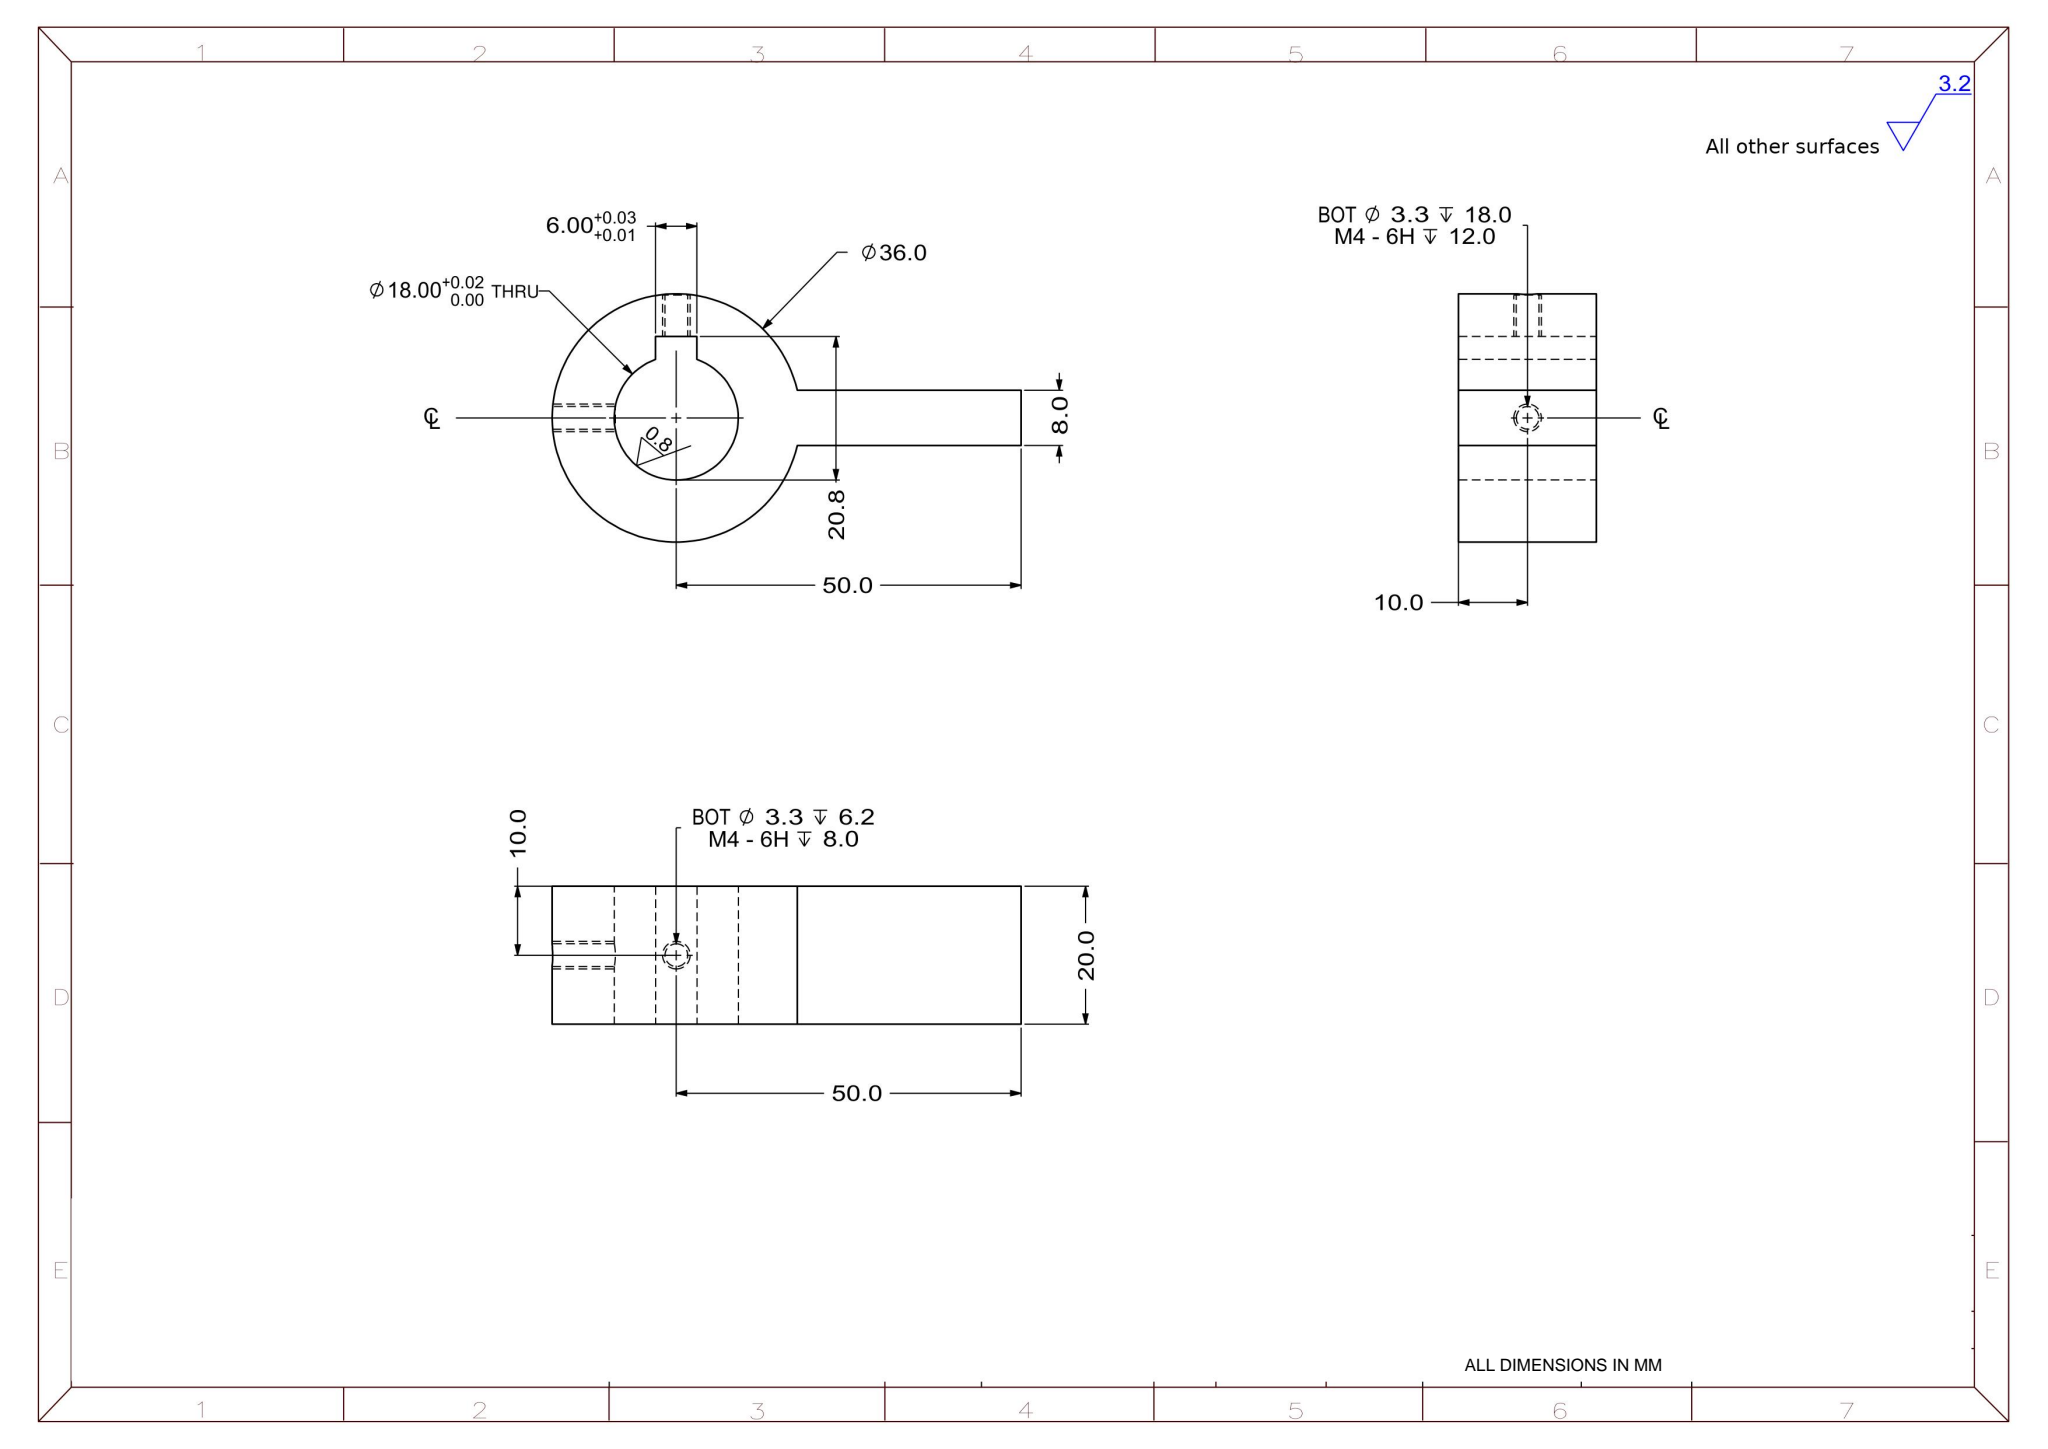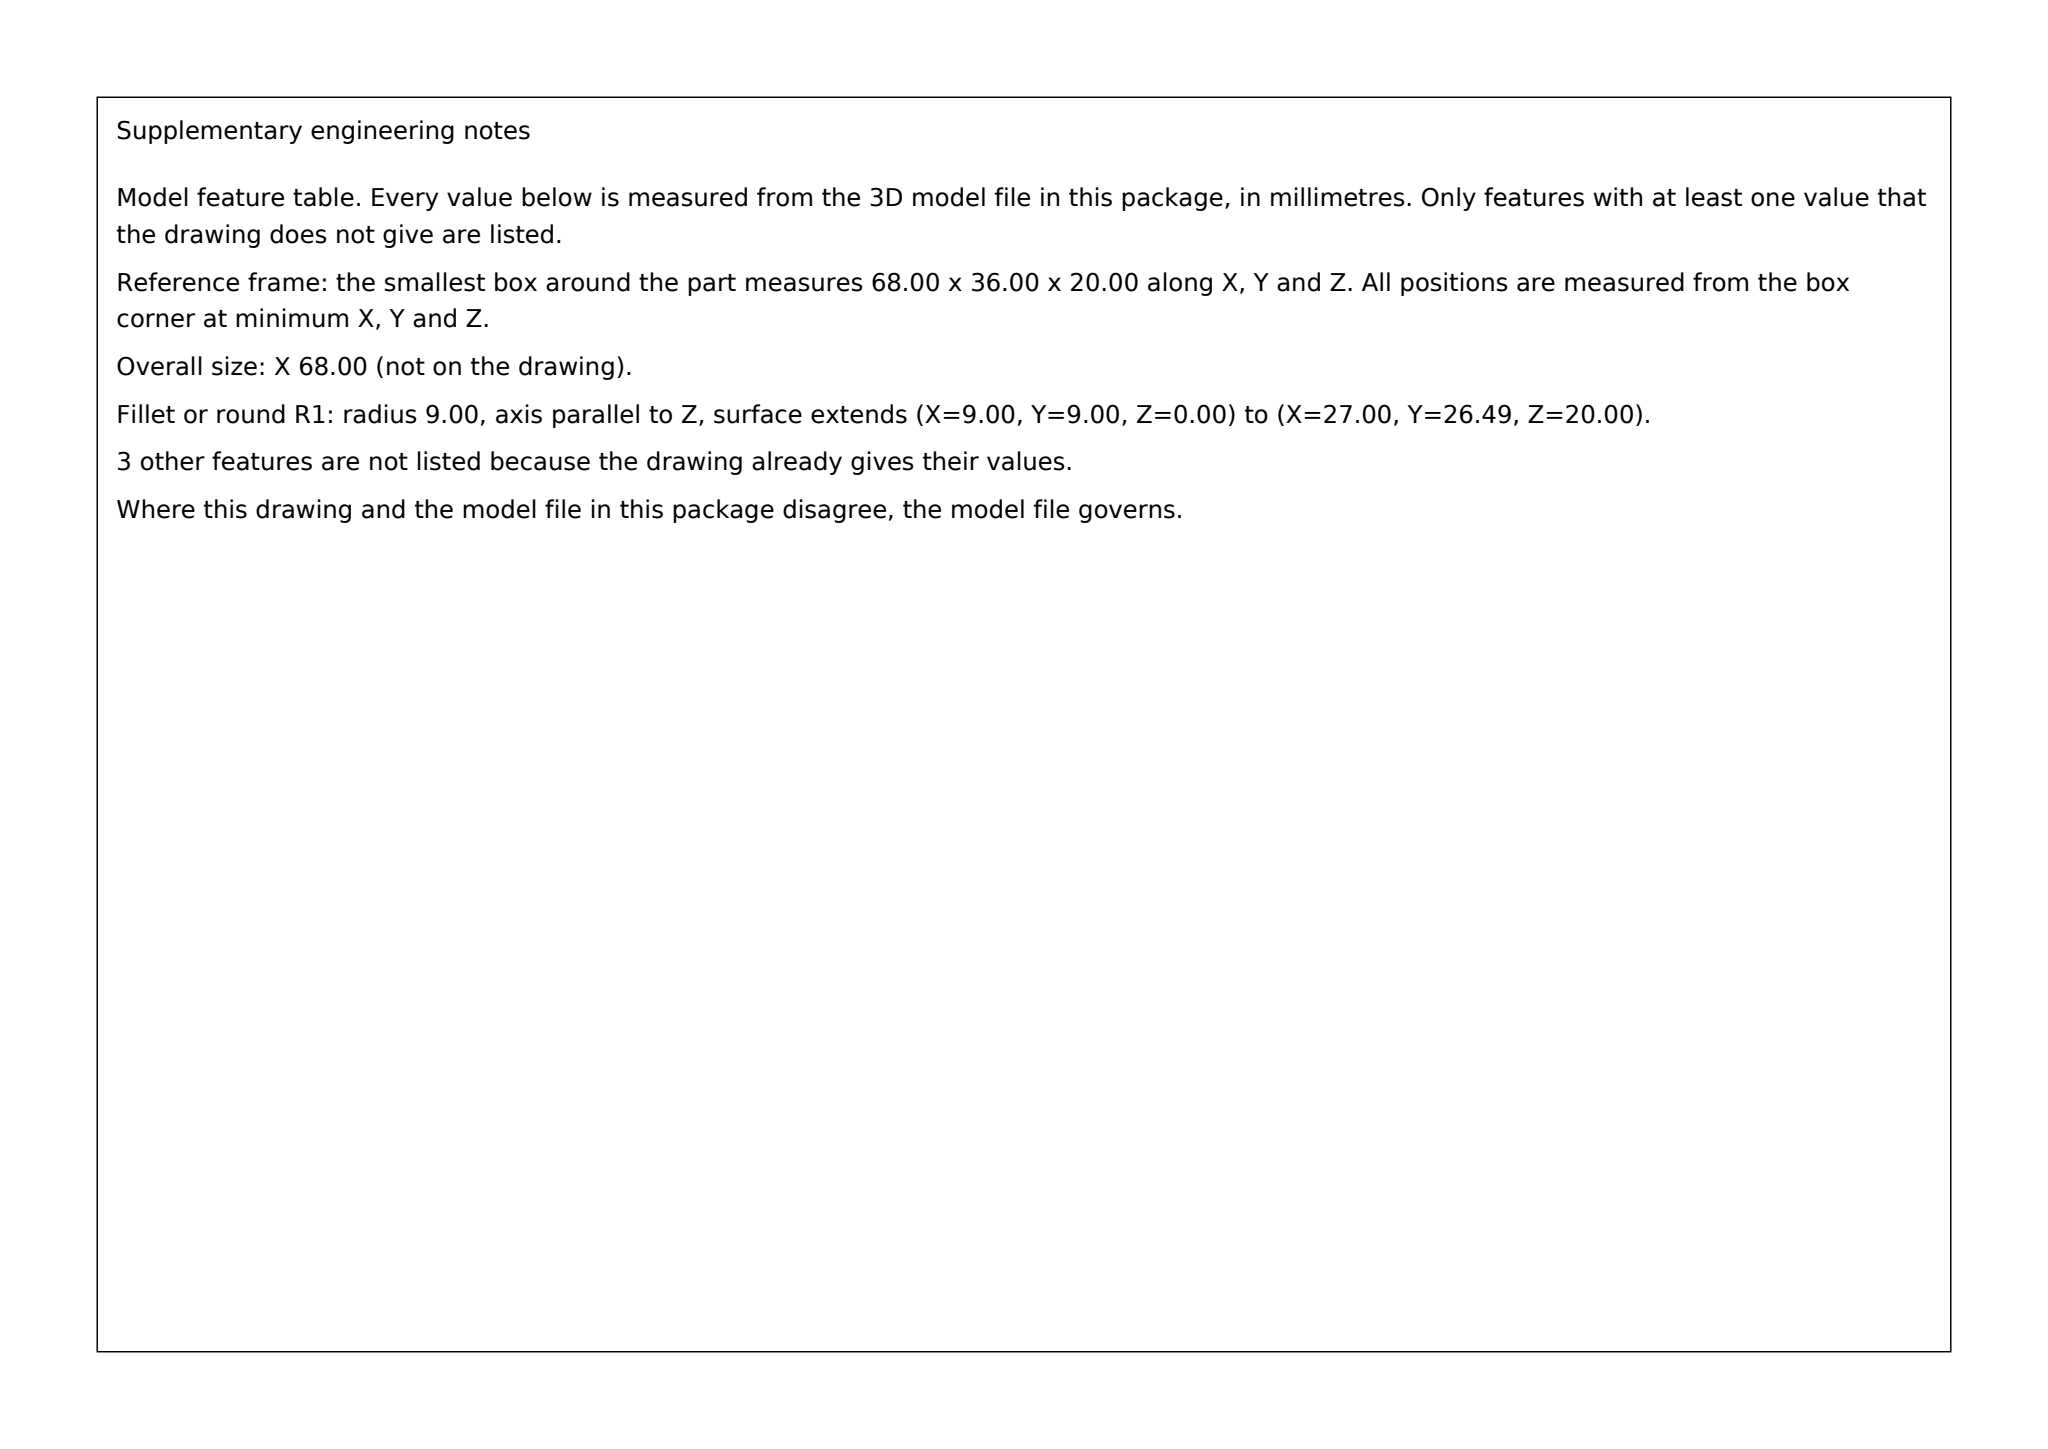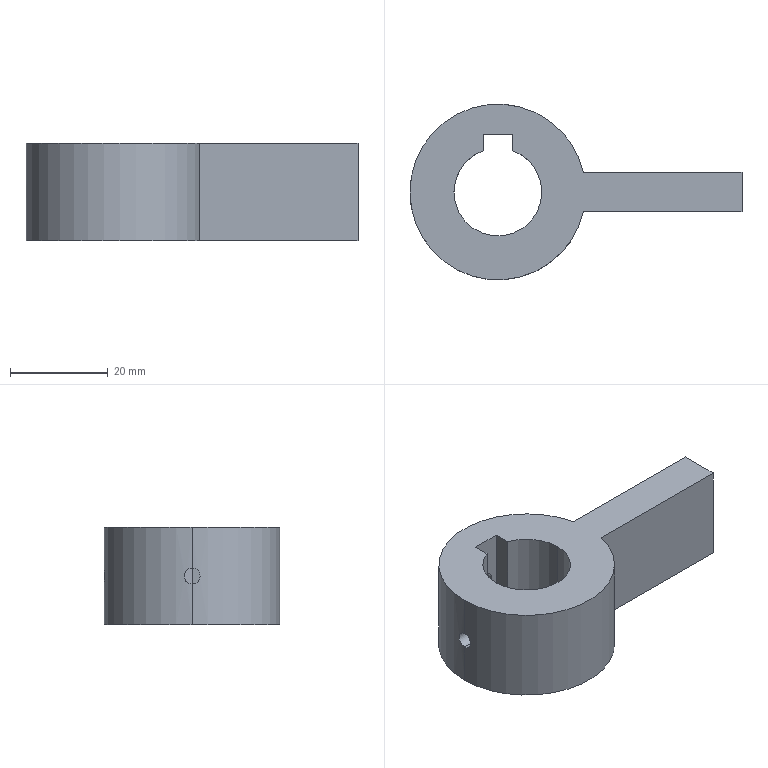Part | SolidWorks | mm | 1 solid | 17 faces | box 68 x 36 x 20 mm | volume 19926 mm3 | cylinder 9 | plane 8 | commonest cylinder face diameters 3.3 x4 18 x3 36 x2
STEP:
#1=CARTESIAN_POINT('',(0.,11.8,1.65));
#2=VERTEX_POINT('',#1);
#3=CARTESIAN_POINT('',(0.,11.8,-1.65));
#4=VERTEX_POINT('',#3);
#5=CARTESIAN_POINT('',(0.,11.8,0.));
#6=DIRECTION('',(0.,-1.,0.));
#7=DIRECTION('',(0.,0.,1.));
#8=AXIS2_PLACEMENT_3D('',#5,#6,#7);
#9=CIRCLE('',#8,1.65);
#10=EDGE_CURVE('',#2,#4,#9,.T.);
#11=ORIENTED_EDGE('',*,*,#10,.T.);
#12=CARTESIAN_POINT('',(0.,18.,-1.65));
#13=VERTEX_POINT('',#12);
#14=CARTESIAN_POINT('',(0.,18.,-1.65));
#15=DIRECTION('',(0.,1.,0.));
#16=VECTOR('',#15,1000.);
#17=LINE('',#14,#16);
#18=EDGE_CURVE('',#4,#13,#17,.T.);
#19=ORIENTED_EDGE('',*,*,#18,.T.);
#20=CARTESIAN_POINT('',(0.,18.,1.65));
#21=VERTEX_POINT('',#20);
#22=CARTESIAN_POINT('',(0.,18.,1.65));
#23=CARTESIAN_POINT('',(-0.1091,18.,1.65));
#24=CARTESIAN_POINT('',(-0.2163,17.999,1.639));
#25=CARTESIAN_POINT('',(-0.4273,17.995,1.597));
#26=CARTESIAN_POINT('',(-0.5321,17.992,1.566));
#27=CARTESIAN_POINT('',(-0.7319,17.985,1.483));
#28=CARTESIAN_POINT('',(-0.8267,17.981,1.432));
#29=CARTESIAN_POINT('',(-1.006,17.972,1.312));
#30=CARTESIAN_POINT('',(-1.091,17.967,1.243));
#31=CARTESIAN_POINT('',(-1.319,17.952,1.014));
#32=CARTESIAN_POINT('',(-1.442,17.942,0.8303));
#33=CARTESIAN_POINT('',(-1.607,17.928,0.4332));
#34=CARTESIAN_POINT('',(-1.65,17.924,0.216));
#35=CARTESIAN_POINT('',(-1.65,17.924,-0.1071));
#36=CARTESIAN_POINT('',(-1.639,17.925,-0.2165));
#37=CARTESIAN_POINT('',(-1.597,17.929,-0.4281));
#38=CARTESIAN_POINT('',(-1.566,17.932,-0.531));
#39=CARTESIAN_POINT('',(-1.483,17.939,-0.7309));
#40=CARTESIAN_POINT('',(-1.432,17.943,-0.8274));
#41=CARTESIAN_POINT('',(-1.312,17.952,-1.006));
#42=CARTESIAN_POINT('',(-1.244,17.957,-1.089));
#43=CARTESIAN_POINT('',(-1.09,17.967,-1.244));
#44=CARTESIAN_POINT('',(-1.007,17.972,-1.312));
#45=CARTESIAN_POINT('',(-0.8279,17.981,-1.431));
#46=CARTESIAN_POINT('',(-0.7314,17.985,-1.483));
#47=CARTESIAN_POINT('',(-0.5315,17.992,-1.566));
#48=CARTESIAN_POINT('',(-0.4287,17.995,-1.597));
#49=CARTESIAN_POINT('',(-0.2171,17.999,-1.639));
#50=CARTESIAN_POINT('',(-0.1077,18.,-1.65));
#51=CARTESIAN_POINT('',(0.,18.,-1.65));
#52=B_SPLINE_CURVE_WITH_KNOTS('',3,(#22,#23,#24,#25,#26,#27,#28,#29,#30,#31,#32,#33,#34,#35,#36,#37,#38,#39,#40,#41,#42,#43,#44,#45,#46,#47,#48,#49,#50,#51),.UNSPECIFIED.,.F.,.F.,(4,2,2,2,2,2,2,2,2,2,2,2,2,2,4),(0.,0.0003226,0.0006452,0.0009678,0.00129,0.001936,0.002581,0.002903,0.003226,0.003548,0.003871,0.004194,0.004516,0.004839,0.005161),.UNSPECIFIED.);
#53=EDGE_CURVE('',#21,#13,#52,.T.);
#54=ORIENTED_EDGE('',*,*,#53,.F.);
#55=CARTESIAN_POINT('',(0.,18.,1.65));
#56=DIRECTION('',(0.,1.,0.));
#57=VECTOR('',#56,1000.);
#58=LINE('',#55,#57);
#59=EDGE_CURVE('',#2,#21,#58,.T.);
#60=ORIENTED_EDGE('',*,*,#59,.F.);
#61=EDGE_LOOP('',(#11,#19,#54,#60));
#62=FACE_OUTER_BOUND('',#61,.T.);
#63=CARTESIAN_POINT('',(0.,18.,0.));
#64=DIRECTION('',(0.,1.,0.));
#65=DIRECTION('',(0.,0.,1.));
#66=AXIS2_PLACEMENT_3D('',#63,#64,#65);
#67=CYLINDRICAL_SURFACE('',#66,1.65);
#68=ADVANCED_FACE('',(#62),#67,.F.);
#69=CARTESIAN_POINT('',(-9.,0.,1.65));
#70=VERTEX_POINT('',#69);
#71=CARTESIAN_POINT('',(-9.,0.,-1.65));
#72=VERTEX_POINT('',#71);
#73=CARTESIAN_POINT('',(-9.,0.,1.65));
#74=CARTESIAN_POINT('',(-9.,-0.1093,1.65));
#75=CARTESIAN_POINT('',(-8.998,-0.2167,1.639));
#76=CARTESIAN_POINT('',(-8.99,-0.4279,1.597));
#77=CARTESIAN_POINT('',(-8.985,-0.5328,1.565));
#78=CARTESIAN_POINT('',(-8.971,-0.7325,1.482));
#79=CARTESIAN_POINT('',(-8.962,-0.8272,1.432));
#80=CARTESIAN_POINT('',(-8.944,-1.006,1.312));
#81=CARTESIAN_POINT('',(-8.934,-1.091,1.242));
#82=CARTESIAN_POINT('',(-8.904,-1.319,1.015));
#83=CARTESIAN_POINT('',(-8.884,-1.442,0.8308));
#84=CARTESIAN_POINT('',(-8.856,-1.606,0.4339));
#85=CARTESIAN_POINT('',(-8.847,-1.65,0.2164));
#86=CARTESIAN_POINT('',(-8.847,-1.65,-0.1072));
#87=CARTESIAN_POINT('',(-8.849,-1.639,-0.2168));
#88=CARTESIAN_POINT('',(-8.857,-1.597,-0.4286));
#89=CARTESIAN_POINT('',(-8.863,-1.566,-0.5316));
#90=CARTESIAN_POINT('',(-8.884,-1.441,-0.8317));
#91=CARTESIAN_POINT('',(-8.904,-1.32,-1.013));
#92=CARTESIAN_POINT('',(-8.934,-1.09,-1.244));
#93=CARTESIAN_POINT('',(-8.944,-1.007,-1.312));
#94=CARTESIAN_POINT('',(-8.962,-0.8283,-1.431));
#95=CARTESIAN_POINT('',(-8.971,-0.7317,-1.483));
#96=CARTESIAN_POINT('',(-8.985,-0.5322,-1.566));
#97=CARTESIAN_POINT('',(-8.99,-0.4293,-1.597));
#98=CARTESIAN_POINT('',(-8.998,-0.2173,-1.639));
#99=CARTESIAN_POINT('',(-9.,-0.1078,-1.65));
#100=CARTESIAN_POINT('',(-9.,0.,-1.65));
#101=B_SPLINE_CURVE_WITH_KNOTS('',3,(#73,#74,#75,#76,#77,#78,#79,#80,#81,#82,#83,#84,#85,#86,#87,#88,#89,#90,#91,#92,#93,#94,#95,#96,#97,#98,#99,#100),.UNSPECIFIED.,.F.,.F.,(4,2,2,2,2,2,2,2,2,2,2,2,2,4),(0.,0.0003231,0.0006462,0.0009693,0.001292,0.001939,0.002585,0.002908,0.003231,0.003877,0.0042,0.004523,0.004846,0.00517),.UNSPECIFIED.);
#102=EDGE_CURVE('',#70,#72,#101,.T.);
#103=ORIENTED_EDGE('',*,*,#102,.T.);
#104=CARTESIAN_POINT('',(-18.,0.,-1.65));
#105=VERTEX_POINT('',#104);
#106=CARTESIAN_POINT('',(-18.,0.,-1.65));
#107=DIRECTION('',(-1.,0.,0.));
#108=VECTOR('',#107,1000.);
#109=LINE('',#106,#108);
#110=EDGE_CURVE('',#72,#105,#109,.T.);
#111=ORIENTED_EDGE('',*,*,#110,.T.);
#112=CARTESIAN_POINT('',(-18.,0.,1.65));
#113=VERTEX_POINT('',#112);
#114=CARTESIAN_POINT('',(-18.,0.,1.65));
#115=CARTESIAN_POINT('',(-18.,-0.1091,1.65));
#116=CARTESIAN_POINT('',(-17.999,-0.2163,1.639));
#117=CARTESIAN_POINT('',(-17.995,-0.4273,1.597));
#118=CARTESIAN_POINT('',(-17.992,-0.5321,1.566));
#119=CARTESIAN_POINT('',(-17.985,-0.7319,1.483));
#120=CARTESIAN_POINT('',(-17.981,-0.8267,1.432));
#121=CARTESIAN_POINT('',(-17.972,-1.006,1.312));
#122=CARTESIAN_POINT('',(-17.967,-1.091,1.243));
#123=CARTESIAN_POINT('',(-17.952,-1.319,1.014));
#124=CARTESIAN_POINT('',(-17.942,-1.442,0.8303));
#125=CARTESIAN_POINT('',(-17.928,-1.607,0.4332));
#126=CARTESIAN_POINT('',(-17.924,-1.65,0.216));
#127=CARTESIAN_POINT('',(-17.924,-1.65,-0.1071));
#128=CARTESIAN_POINT('',(-17.925,-1.639,-0.2165));
#129=CARTESIAN_POINT('',(-17.929,-1.597,-0.4281));
#130=CARTESIAN_POINT('',(-17.932,-1.566,-0.531));
#131=CARTESIAN_POINT('',(-17.939,-1.483,-0.7309));
#132=CARTESIAN_POINT('',(-17.943,-1.432,-0.8274));
#133=CARTESIAN_POINT('',(-17.952,-1.312,-1.006));
#134=CARTESIAN_POINT('',(-17.957,-1.244,-1.089));
#135=CARTESIAN_POINT('',(-17.967,-1.09,-1.244));
#136=CARTESIAN_POINT('',(-17.972,-1.007,-1.312));
#137=CARTESIAN_POINT('',(-17.981,-0.8279,-1.431));
#138=CARTESIAN_POINT('',(-17.985,-0.7314,-1.483));
#139=CARTESIAN_POINT('',(-17.992,-0.5315,-1.566));
#140=CARTESIAN_POINT('',(-17.995,-0.4287,-1.597));
#141=CARTESIAN_POINT('',(-17.999,-0.2171,-1.639));
#142=CARTESIAN_POINT('',(-18.,-0.1077,-1.65));
#143=CARTESIAN_POINT('',(-18.,0.,-1.65));
#144=B_SPLINE_CURVE_WITH_KNOTS('',3,(#114,#115,#116,#117,#118,#119,#120,#121,#122,#123,#124,#125,#126,#127,#128,#129,#130,#131,#132,#133,#134,#135,#136,#137,#138,#139,#140,#141,#142,#143),.UNSPECIFIED.,.F.,.F.,(4,2,2,2,2,2,2,2,2,2,2,2,2,2,4),(0.,0.0003226,0.0006452,0.0009678,0.00129,0.001936,0.002581,0.002903,0.003226,0.003548,0.003871,0.004194,0.004516,0.004839,0.005161),.UNSPECIFIED.);
#145=EDGE_CURVE('',#113,#105,#144,.T.);
#146=ORIENTED_EDGE('',*,*,#145,.F.);
#147=CARTESIAN_POINT('',(-18.,0.,1.65));
#148=DIRECTION('',(-1.,0.,0.));
#149=VECTOR('',#148,1000.);
#150=LINE('',#147,#149);
#151=EDGE_CURVE('',#70,#113,#150,.T.);
#152=ORIENTED_EDGE('',*,*,#151,.F.);
#153=EDGE_LOOP('',(#103,#111,#146,#152));
#154=FACE_OUTER_BOUND('',#153,.T.);
#155=CARTESIAN_POINT('',(-18.,0.,0.));
#156=DIRECTION('',(-1.,0.,0.));
#157=DIRECTION('',(0.,0.,1.));
#158=AXIS2_PLACEMENT_3D('',#155,#156,#157);
#159=CYLINDRICAL_SURFACE('',#158,1.65);
#160=ADVANCED_FACE('',(#154),#159,.F.);
#161=CARTESIAN_POINT('',(-9.,0.,10.));
#162=VERTEX_POINT('',#161);
#163=CARTESIAN_POINT('',(9.,0.,10.));
#164=VERTEX_POINT('',#163);
#165=CARTESIAN_POINT('',(0.,0.,10.));
#166=DIRECTION('',(0.,0.,1.));
#167=DIRECTION('',(1.,0.,0.));
#168=AXIS2_PLACEMENT_3D('',#165,#166,#167);
#169=CIRCLE('',#168,9.);
#170=EDGE_CURVE('',#162,#164,#169,.T.);
#171=ORIENTED_EDGE('',*,*,#170,.T.);
#172=CARTESIAN_POINT('',(9.,0.,-10.));
#173=VERTEX_POINT('',#172);
#174=CARTESIAN_POINT('',(9.,0.,10.));
#175=DIRECTION('',(0.,0.,-1.));
#176=VECTOR('',#175,1000.);
#177=LINE('',#174,#176);
#178=EDGE_CURVE('',#164,#173,#177,.T.);
#179=ORIENTED_EDGE('',*,*,#178,.T.);
#180=CARTESIAN_POINT('',(-9.,0.,-10.));
#181=VERTEX_POINT('',#180);
#182=CARTESIAN_POINT('',(0.,0.,-10.));
#183=DIRECTION('',(0.,0.,1.));
#184=DIRECTION('',(1.,0.,0.));
#185=AXIS2_PLACEMENT_3D('',#182,#183,#184);
#186=CIRCLE('',#185,9.);
#187=EDGE_CURVE('',#181,#173,#186,.T.);
#188=ORIENTED_EDGE('',*,*,#187,.F.);
#189=CARTESIAN_POINT('',(-9.,0.,10.));
#190=DIRECTION('',(0.,0.,-1.));
#191=VECTOR('',#190,1000.);
#192=LINE('',#189,#191);
#193=EDGE_CURVE('',#72,#181,#192,.T.);
#194=ORIENTED_EDGE('',*,*,#193,.F.);
#195=ORIENTED_EDGE('',*,*,#102,.F.);
#196=CARTESIAN_POINT('',(-9.,0.,10.));
#197=DIRECTION('',(0.,0.,-1.));
#198=VECTOR('',#197,1000.);
#199=LINE('',#196,#198);
#200=EDGE_CURVE('',#162,#70,#199,.T.);
#201=ORIENTED_EDGE('',*,*,#200,.F.);
#202=EDGE_LOOP('',(#171,#179,#188,#194,#195,#201));
#203=FACE_OUTER_BOUND('',#202,.T.);
#204=CARTESIAN_POINT('',(0.,0.,10.));
#205=DIRECTION('',(0.,0.,-1.));
#206=DIRECTION('',(-1.,0.,0.));
#207=AXIS2_PLACEMENT_3D('',#204,#205,#206);
#208=CYLINDRICAL_SURFACE('',#207,9.);
#209=ADVANCED_FACE('',(#203),#208,.F.);
#210=CARTESIAN_POINT('',(-3.,8.485,10.));
#211=VERTEX_POINT('',#210);
#212=CARTESIAN_POINT('',(0.,0.,10.));
#213=DIRECTION('',(0.,0.,1.));
#214=DIRECTION('',(1.,0.,0.));
#215=AXIS2_PLACEMENT_3D('',#212,#213,#214);
#216=CIRCLE('',#215,9.);
#217=EDGE_CURVE('',#211,#162,#216,.T.);
#218=ORIENTED_EDGE('',*,*,#217,.T.);
#219=ORIENTED_EDGE('',*,*,#200,.T.);
#220=CARTESIAN_POINT('',(-9.,0.,-1.65));
#221=CARTESIAN_POINT('',(-9.,0.2156,-1.65));
#222=CARTESIAN_POINT('',(-8.992,0.4331,-1.607));
#223=CARTESIAN_POINT('',(-8.964,0.8303,-1.442));
#224=CARTESIAN_POINT('',(-8.944,1.014,-1.319));
#225=CARTESIAN_POINT('',(-8.914,1.242,-1.091));
#226=CARTESIAN_POINT('',(-8.904,1.312,-1.007));
#227=CARTESIAN_POINT('',(-8.886,1.431,-0.828));
#228=CARTESIAN_POINT('',(-8.877,1.482,-0.7334));
#229=CARTESIAN_POINT('',(-8.856,1.607,-0.4333));
#230=CARTESIAN_POINT('',(-8.847,1.65,-0.2189));
#231=CARTESIAN_POINT('',(-8.847,1.65,0.1081));
#232=CARTESIAN_POINT('',(-8.849,1.639,0.2153));
#233=CARTESIAN_POINT('',(-8.857,1.598,0.4267));
#234=CARTESIAN_POINT('',(-8.863,1.566,0.5318));
#235=CARTESIAN_POINT('',(-8.877,1.483,0.7312));
#236=CARTESIAN_POINT('',(-8.885,1.432,0.826));
#237=CARTESIAN_POINT('',(-8.904,1.313,1.006));
#238=CARTESIAN_POINT('',(-8.914,1.243,1.09));
#239=CARTESIAN_POINT('',(-8.944,1.016,1.318));
#240=CARTESIAN_POINT('',(-8.964,0.8322,1.441));
#241=CARTESIAN_POINT('',(-8.992,0.4354,1.606));
#242=CARTESIAN_POINT('',(-9.,0.2185,1.65));
#243=CARTESIAN_POINT('',(-9.,0.,1.65));
#244=B_SPLINE_CURVE_WITH_KNOTS('',3,(#220,#221,#222,#223,#224,#225,#226,#227,#228,#229,#230,#231,#232,#233,#234,#235,#236,#237,#238,#239,#240,#241,#242,#243),.UNSPECIFIED.,.F.,.F.,(4,2,2,2,2,2,2,2,2,2,2,4),(0.00517,0.005816,0.006462,0.006785,0.007108,0.007754,0.008077,0.0084,0.008723,0.009046,0.009692,0.01034),.UNSPECIFIED.);
#245=EDGE_CURVE('',#72,#70,#244,.T.);
#246=ORIENTED_EDGE('',*,*,#245,.F.);
#247=ORIENTED_EDGE('',*,*,#193,.T.);
#248=CARTESIAN_POINT('',(-3.,8.485,-10.));
#249=VERTEX_POINT('',#248);
#250=CARTESIAN_POINT('',(0.,0.,-10.));
#251=DIRECTION('',(0.,0.,1.));
#252=DIRECTION('',(1.,0.,0.));
#253=AXIS2_PLACEMENT_3D('',#250,#251,#252);
#254=CIRCLE('',#253,9.);
#255=EDGE_CURVE('',#249,#181,#254,.T.);
#256=ORIENTED_EDGE('',*,*,#255,.F.);
#257=CARTESIAN_POINT('',(-3.,8.485,10.));
#258=DIRECTION('',(0.,0.,-1.));
#259=VECTOR('',#258,1000.);
#260=LINE('',#257,#259);
#261=EDGE_CURVE('',#211,#249,#260,.T.);
#262=ORIENTED_EDGE('',*,*,#261,.F.);
#263=EDGE_LOOP('',(#218,#219,#246,#247,#256,#262));
#264=FACE_OUTER_BOUND('',#263,.T.);
#265=CARTESIAN_POINT('',(0.,0.,10.));
#266=DIRECTION('',(0.,0.,-1.));
#267=DIRECTION('',(-1.,0.,0.));
#268=AXIS2_PLACEMENT_3D('',#265,#266,#267);
#269=CYLINDRICAL_SURFACE('',#268,9.);
#270=ADVANCED_FACE('',(#264),#269,.F.);
#271=CARTESIAN_POINT('',(-18.,0.,10.));
#272=VERTEX_POINT('',#271);
#273=CARTESIAN_POINT('',(17.55,-4.,10.));
#274=VERTEX_POINT('',#273);
#275=CARTESIAN_POINT('',(0.,0.,10.));
#276=DIRECTION('',(0.,0.,1.));
#277=DIRECTION('',(1.,0.,0.));
#278=AXIS2_PLACEMENT_3D('',#275,#276,#277);
#279=CIRCLE('',#278,18.);
#280=EDGE_CURVE('',#272,#274,#279,.T.);
#281=ORIENTED_EDGE('',*,*,#280,.F.);
#282=CARTESIAN_POINT('',(-18.,0.,10.));
#283=DIRECTION('',(0.,0.,-1.));
#284=VECTOR('',#283,1000.);
#285=LINE('',#282,#284);
#286=EDGE_CURVE('',#272,#113,#285,.T.);
#287=ORIENTED_EDGE('',*,*,#286,.T.);
#288=ORIENTED_EDGE('',*,*,#145,.T.);
#289=CARTESIAN_POINT('',(-18.,0.,-10.));
#290=VERTEX_POINT('',#289);
#291=CARTESIAN_POINT('',(-18.,0.,10.));
#292=DIRECTION('',(0.,0.,-1.));
#293=VECTOR('',#292,1000.);
#294=LINE('',#291,#293);
#295=EDGE_CURVE('',#105,#290,#294,.T.);
#296=ORIENTED_EDGE('',*,*,#295,.T.);
#297=CARTESIAN_POINT('',(17.55,-4.,-10.));
#298=VERTEX_POINT('',#297);
#299=CARTESIAN_POINT('',(0.,0.,-10.));
#300=DIRECTION('',(0.,0.,1.));
#301=DIRECTION('',(1.,0.,0.));
#302=AXIS2_PLACEMENT_3D('',#299,#300,#301);
#303=CIRCLE('',#302,18.);
#304=EDGE_CURVE('',#290,#298,#303,.T.);
#305=ORIENTED_EDGE('',*,*,#304,.T.);
#306=CARTESIAN_POINT('',(17.55,-4.,10.));
#307=DIRECTION('',(0.,0.,-1.));
#308=VECTOR('',#307,1000.);
#309=LINE('',#306,#308);
#310=EDGE_CURVE('',#274,#298,#309,.T.);
#311=ORIENTED_EDGE('',*,*,#310,.F.);
#312=EDGE_LOOP('',(#281,#287,#288,#296,#305,#311));
#313=FACE_OUTER_BOUND('',#312,.T.);
#314=CARTESIAN_POINT('',(0.,0.,10.));
#315=DIRECTION('',(0.,0.,-1.));
#316=DIRECTION('',(-1.,0.,0.));
#317=AXIS2_PLACEMENT_3D('',#314,#315,#316);
#318=CYLINDRICAL_SURFACE('',#317,18.);
#319=ADVANCED_FACE('',(#313),#318,.T.);
#320=CARTESIAN_POINT('',(17.55,4.,-10.));
#321=VERTEX_POINT('',#320);
#322=CARTESIAN_POINT('',(50.,4.,-10.));
#323=VERTEX_POINT('',#322);
#324=CARTESIAN_POINT('',(0.,4.,-10.));
#325=DIRECTION('',(1.,0.,0.));
#326=VECTOR('',#325,1000.);
#327=LINE('',#324,#326);
#328=EDGE_CURVE('',#321,#323,#327,.T.);
#329=ORIENTED_EDGE('',*,*,#328,.F.);
#330=CARTESIAN_POINT('',(17.55,4.,10.));
#331=VERTEX_POINT('',#330);
#332=CARTESIAN_POINT('',(17.55,4.,10.));
#333=DIRECTION('',(0.,0.,-1.));
#334=VECTOR('',#333,1000.);
#335=LINE('',#332,#334);
#336=EDGE_CURVE('',#331,#321,#335,.T.);
#337=ORIENTED_EDGE('',*,*,#336,.F.);
#338=CARTESIAN_POINT('',(50.,4.,10.));
#339=VERTEX_POINT('',#338);
#340=CARTESIAN_POINT('',(0.,4.,10.));
#341=DIRECTION('',(1.,0.,0.));
#342=VECTOR('',#341,1000.);
#343=LINE('',#340,#342);
#344=EDGE_CURVE('',#331,#339,#343,.T.);
#345=ORIENTED_EDGE('',*,*,#344,.T.);
#346=CARTESIAN_POINT('',(50.,4.,10.));
#347=DIRECTION('',(0.,0.,-1.));
#348=VECTOR('',#347,1000.);
#349=LINE('',#346,#348);
#350=EDGE_CURVE('',#339,#323,#349,.T.);
#351=ORIENTED_EDGE('',*,*,#350,.T.);
#352=EDGE_LOOP('',(#329,#337,#345,#351));
#353=FACE_OUTER_BOUND('',#352,.T.);
#354=CARTESIAN_POINT('',(0.,4.,10.));
#355=DIRECTION('',(0.,1.,0.));
#356=DIRECTION('',(0.,0.,1.));
#357=AXIS2_PLACEMENT_3D('',#354,#355,#356);
#358=PLANE('',#357);
#359=ADVANCED_FACE('',(#353),#358,.T.);
#360=ORIENTED_EDGE('',*,*,#286,.F.);
#361=CARTESIAN_POINT('',(0.,0.,10.));
#362=DIRECTION('',(0.,0.,1.));
#363=DIRECTION('',(1.,0.,0.));
#364=AXIS2_PLACEMENT_3D('',#361,#362,#363);
#365=CIRCLE('',#364,18.);
#366=EDGE_CURVE('',#331,#272,#365,.T.);
#367=ORIENTED_EDGE('',*,*,#366,.F.);
#368=ORIENTED_EDGE('',*,*,#336,.T.);
#369=CARTESIAN_POINT('',(0.,0.,-10.));
#370=DIRECTION('',(0.,0.,1.));
#371=DIRECTION('',(1.,0.,0.));
#372=AXIS2_PLACEMENT_3D('',#369,#370,#371);
#373=CIRCLE('',#372,18.);
#374=EDGE_CURVE('',#321,#290,#373,.T.);
#375=ORIENTED_EDGE('',*,*,#374,.T.);
#376=ORIENTED_EDGE('',*,*,#295,.F.);
#377=CARTESIAN_POINT('',(-18.,0.,-1.65));
#378=CARTESIAN_POINT('',(-18.,0.2154,-1.65));
#379=CARTESIAN_POINT('',(-17.996,0.4325,-1.607));
#380=CARTESIAN_POINT('',(-17.982,0.8297,-1.442));
#381=CARTESIAN_POINT('',(-17.972,1.014,-1.32));
#382=CARTESIAN_POINT('',(-17.957,1.242,-1.092));
#383=CARTESIAN_POINT('',(-17.952,1.312,-1.007));
#384=CARTESIAN_POINT('',(-17.943,1.432,-0.8275));
#385=CARTESIAN_POINT('',(-17.939,1.482,-0.7328));
#386=CARTESIAN_POINT('',(-17.932,1.565,-0.5332));
#387=CARTESIAN_POINT('',(-17.929,1.597,-0.4283));
#388=CARTESIAN_POINT('',(-17.925,1.639,-0.2174));
#389=CARTESIAN_POINT('',(-17.924,1.65,-0.1103));
#390=CARTESIAN_POINT('',(-17.924,1.65,0.1077));
#391=CARTESIAN_POINT('',(-17.925,1.639,0.2151));
#392=CARTESIAN_POINT('',(-17.929,1.598,0.4261));
#393=CARTESIAN_POINT('',(-17.932,1.566,0.5308));
#394=CARTESIAN_POINT('',(-17.939,1.483,0.7307));
#395=CARTESIAN_POINT('',(-17.943,1.433,0.8255));
#396=CARTESIAN_POINT('',(-17.952,1.313,1.005));
#397=CARTESIAN_POINT('',(-17.957,1.244,1.09));
#398=CARTESIAN_POINT('',(-17.972,1.015,1.318));
#399=CARTESIAN_POINT('',(-17.982,0.8317,1.441));
#400=CARTESIAN_POINT('',(-17.996,0.4348,1.606));
#401=CARTESIAN_POINT('',(-18.,0.2181,1.65));
#402=CARTESIAN_POINT('',(-18.,0.,1.65));
#403=B_SPLINE_CURVE_WITH_KNOTS('',3,(#377,#378,#379,#380,#381,#382,#383,#384,#385,#386,#387,#388,#389,#390,#391,#392,#393,#394,#395,#396,#397,#398,#399,#400,#401,#402),.UNSPECIFIED.,.F.,.F.,(4,2,2,2,2,2,2,2,2,2,2,2,4),(0.005161,0.005806,0.006451,0.006774,0.007096,0.007419,0.007741,0.008064,0.008386,0.008709,0.009031,0.009676,0.01032),.UNSPECIFIED.);
#404=EDGE_CURVE('',#105,#113,#403,.T.);
#405=ORIENTED_EDGE('',*,*,#404,.T.);
#406=EDGE_LOOP('',(#360,#367,#368,#375,#376,#405));
#407=FACE_OUTER_BOUND('',#406,.T.);
#408=ORIENTED_EDGE('',*,*,#53,.T.);
#409=CARTESIAN_POINT('',(0.,18.,-1.65));
#410=CARTESIAN_POINT('',(0.2154,18.,-1.65));
#411=CARTESIAN_POINT('',(0.4325,17.996,-1.607));
#412=CARTESIAN_POINT('',(0.8297,17.982,-1.442));
#413=CARTESIAN_POINT('',(1.014,17.972,-1.32));
#414=CARTESIAN_POINT('',(1.242,17.957,-1.092));
#415=CARTESIAN_POINT('',(1.312,17.952,-1.007));
#416=CARTESIAN_POINT('',(1.432,17.943,-0.8275));
#417=CARTESIAN_POINT('',(1.482,17.939,-0.7328));
#418=CARTESIAN_POINT('',(1.565,17.932,-0.5332));
#419=CARTESIAN_POINT('',(1.597,17.929,-0.4283));
#420=CARTESIAN_POINT('',(1.639,17.925,-0.2174));
#421=CARTESIAN_POINT('',(1.65,17.924,-0.1103));
#422=CARTESIAN_POINT('',(1.65,17.924,0.1077));
#423=CARTESIAN_POINT('',(1.639,17.925,0.2151));
#424=CARTESIAN_POINT('',(1.598,17.929,0.4261));
#425=CARTESIAN_POINT('',(1.566,17.932,0.5308));
#426=CARTESIAN_POINT('',(1.483,17.939,0.7307));
#427=CARTESIAN_POINT('',(1.433,17.943,0.8255));
#428=CARTESIAN_POINT('',(1.313,17.952,1.005));
#429=CARTESIAN_POINT('',(1.244,17.957,1.09));
#430=CARTESIAN_POINT('',(1.015,17.972,1.318));
#431=CARTESIAN_POINT('',(0.8317,17.982,1.441));
#432=CARTESIAN_POINT('',(0.4348,17.996,1.606));
#433=CARTESIAN_POINT('',(0.2181,18.,1.65));
#434=CARTESIAN_POINT('',(0.,18.,1.65));
#435=B_SPLINE_CURVE_WITH_KNOTS('',3,(#409,#410,#411,#412,#413,#414,#415,#416,#417,#418,#419,#420,#421,#422,#423,#424,#425,#426,#427,#428,#429,#430,#431,#432,#433,#434),.UNSPECIFIED.,.F.,.F.,(4,2,2,2,2,2,2,2,2,2,2,2,4),(0.005161,0.005806,0.006451,0.006774,0.007096,0.007419,0.007741,0.008064,0.008386,0.008709,0.009031,0.009676,0.01032),.UNSPECIFIED.);
#436=EDGE_CURVE('',#13,#21,#435,.T.);
#437=ORIENTED_EDGE('',*,*,#436,.T.);
#438=EDGE_LOOP('',(#408,#437));
#439=FACE_BOUND('',#438,.T.);
#440=CARTESIAN_POINT('',(0.,0.,10.));
#441=DIRECTION('',(0.,0.,-1.));
#442=DIRECTION('',(-1.,0.,0.));
#443=AXIS2_PLACEMENT_3D('',#440,#441,#442);
#444=CYLINDRICAL_SURFACE('',#443,18.);
#445=ADVANCED_FACE('',(#407,#439),#444,.T.);
#446=CARTESIAN_POINT('',(50.,-4.,-10.));
#447=VERTEX_POINT('',#446);
#448=CARTESIAN_POINT('',(0.,-4.,-10.));
#449=DIRECTION('',(1.,0.,0.));
#450=VECTOR('',#449,1000.);
#451=LINE('',#448,#450);
#452=EDGE_CURVE('',#298,#447,#451,.T.);
#453=ORIENTED_EDGE('',*,*,#452,.T.);
#454=CARTESIAN_POINT('',(50.,-4.,10.));
#455=VERTEX_POINT('',#454);
#456=CARTESIAN_POINT('',(50.,-4.,10.));
#457=DIRECTION('',(0.,0.,-1.));
#458=VECTOR('',#457,1000.);
#459=LINE('',#456,#458);
#460=EDGE_CURVE('',#455,#447,#459,.T.);
#461=ORIENTED_EDGE('',*,*,#460,.F.);
#462=CARTESIAN_POINT('',(0.,-4.,10.));
#463=DIRECTION('',(1.,0.,0.));
#464=VECTOR('',#463,1000.);
#465=LINE('',#462,#464);
#466=EDGE_CURVE('',#274,#455,#465,.T.);
#467=ORIENTED_EDGE('',*,*,#466,.F.);
#468=ORIENTED_EDGE('',*,*,#310,.T.);
#469=EDGE_LOOP('',(#453,#461,#467,#468));
#470=FACE_OUTER_BOUND('',#469,.T.);
#471=CARTESIAN_POINT('',(0.,-4.,10.));
#472=DIRECTION('',(0.,1.,0.));
#473=DIRECTION('',(0.,0.,1.));
#474=AXIS2_PLACEMENT_3D('',#471,#472,#473);
#475=PLANE('',#474);
#476=ADVANCED_FACE('',(#470),#475,.F.);
#477=CARTESIAN_POINT('',(3.,8.485,-10.));
#478=VERTEX_POINT('',#477);
#479=CARTESIAN_POINT('',(3.,11.8,-10.));
#480=VERTEX_POINT('',#479);
#481=CARTESIAN_POINT('',(3.,-0.,-10.));
#482=DIRECTION('',(0.,1.,0.));
#483=VECTOR('',#482,1000.);
#484=LINE('',#481,#483);
#485=EDGE_CURVE('',#478,#480,#484,.T.);
#486=ORIENTED_EDGE('',*,*,#485,.F.);
#487=CARTESIAN_POINT('',(3.,8.485,10.));
#488=VERTEX_POINT('',#487);
#489=CARTESIAN_POINT('',(3.,8.485,10.));
#490=DIRECTION('',(0.,0.,-1.));
#491=VECTOR('',#490,1000.);
#492=LINE('',#489,#491);
#493=EDGE_CURVE('',#488,#478,#492,.T.);
#494=ORIENTED_EDGE('',*,*,#493,.F.);
#495=CARTESIAN_POINT('',(3.,11.8,10.));
#496=VERTEX_POINT('',#495);
#497=CARTESIAN_POINT('',(3.,-0.,10.));
#498=DIRECTION('',(0.,1.,0.));
#499=VECTOR('',#498,1000.);
#500=LINE('',#497,#499);
#501=EDGE_CURVE('',#488,#496,#500,.T.);
#502=ORIENTED_EDGE('',*,*,#501,.T.);
#503=CARTESIAN_POINT('',(3.,11.8,10.));
#504=DIRECTION('',(0.,0.,-1.));
#505=VECTOR('',#504,1000.);
#506=LINE('',#503,#505);
#507=EDGE_CURVE('',#496,#480,#506,.T.);
#508=ORIENTED_EDGE('',*,*,#507,.T.);
#509=EDGE_LOOP('',(#486,#494,#502,#508));
#510=FACE_OUTER_BOUND('',#509,.T.);
#511=CARTESIAN_POINT('',(3.,-0.,10.));
#512=DIRECTION('',(-1.,0.,0.));
#513=DIRECTION('',(-0.,-1.,0.));
#514=AXIS2_PLACEMENT_3D('',#511,#512,#513);
#515=PLANE('',#514);
#516=ADVANCED_FACE('',(#510),#515,.T.);
#517=ORIENTED_EDGE('',*,*,#178,.F.);
#518=CARTESIAN_POINT('',(0.,0.,10.));
#519=DIRECTION('',(0.,0.,1.));
#520=DIRECTION('',(1.,0.,0.));
#521=AXIS2_PLACEMENT_3D('',#518,#519,#520);
#522=CIRCLE('',#521,9.);
#523=EDGE_CURVE('',#164,#488,#522,.T.);
#524=ORIENTED_EDGE('',*,*,#523,.T.);
#525=ORIENTED_EDGE('',*,*,#493,.T.);
#526=CARTESIAN_POINT('',(0.,0.,-10.));
#527=DIRECTION('',(0.,0.,1.));
#528=DIRECTION('',(1.,0.,0.));
#529=AXIS2_PLACEMENT_3D('',#526,#527,#528);
#530=CIRCLE('',#529,9.);
#531=EDGE_CURVE('',#173,#478,#530,.T.);
#532=ORIENTED_EDGE('',*,*,#531,.F.);
#533=EDGE_LOOP('',(#517,#524,#525,#532));
#534=FACE_OUTER_BOUND('',#533,.T.);
#535=CARTESIAN_POINT('',(0.,0.,10.));
#536=DIRECTION('',(0.,0.,-1.));
#537=DIRECTION('',(-1.,0.,0.));
#538=AXIS2_PLACEMENT_3D('',#535,#536,#537);
#539=CYLINDRICAL_SURFACE('',#538,9.);
#540=ADVANCED_FACE('',(#534),#539,.F.);
#541=CARTESIAN_POINT('',(-3.,11.8,-10.));
#542=VERTEX_POINT('',#541);
#543=CARTESIAN_POINT('',(-3.,0.,-10.));
#544=DIRECTION('',(0.,1.,0.));
#545=VECTOR('',#544,1000.);
#546=LINE('',#543,#545);
#547=EDGE_CURVE('',#249,#542,#546,.T.);
#548=ORIENTED_EDGE('',*,*,#547,.T.);
#549=CARTESIAN_POINT('',(-3.,11.8,10.));
#550=VERTEX_POINT('',#549);
#551=CARTESIAN_POINT('',(-3.,11.8,10.));
#552=DIRECTION('',(0.,0.,-1.));
#553=VECTOR('',#552,1000.);
#554=LINE('',#551,#553);
#555=EDGE_CURVE('',#550,#542,#554,.T.);
#556=ORIENTED_EDGE('',*,*,#555,.F.);
#557=CARTESIAN_POINT('',(-3.,0.,10.));
#558=DIRECTION('',(0.,1.,0.));
#559=VECTOR('',#558,1000.);
#560=LINE('',#557,#559);
#561=EDGE_CURVE('',#211,#550,#560,.T.);
#562=ORIENTED_EDGE('',*,*,#561,.F.);
#563=ORIENTED_EDGE('',*,*,#261,.T.);
#564=EDGE_LOOP('',(#548,#556,#562,#563));
#565=FACE_OUTER_BOUND('',#564,.T.);
#566=CARTESIAN_POINT('',(-3.,0.,10.));
#567=DIRECTION('',(-1.,0.,0.));
#568=DIRECTION('',(-0.,-1.,0.));
#569=AXIS2_PLACEMENT_3D('',#566,#567,#568);
#570=PLANE('',#569);
#571=ADVANCED_FACE('',(#565),#570,.F.);
#572=ORIENTED_EDGE('',*,*,#10,.F.);
#573=CARTESIAN_POINT('',(0.,11.8,0.));
#574=DIRECTION('',(0.,-1.,0.));
#575=DIRECTION('',(0.,0.,1.));
#576=AXIS2_PLACEMENT_3D('',#573,#574,#575);
#577=CIRCLE('',#576,1.65);
#578=EDGE_CURVE('',#4,#2,#577,.T.);
#579=ORIENTED_EDGE('',*,*,#578,.F.);
#580=EDGE_LOOP('',(#572,#579));
#581=FACE_BOUND('',#580,.T.);
#582=CARTESIAN_POINT('',(0.,11.8,-10.));
#583=DIRECTION('',(1.,0.,0.));
#584=VECTOR('',#583,1000.);
#585=LINE('',#582,#584);
#586=EDGE_CURVE('',#542,#480,#585,.T.);
#587=ORIENTED_EDGE('',*,*,#586,.T.);
#588=ORIENTED_EDGE('',*,*,#507,.F.);
#589=CARTESIAN_POINT('',(0.,11.8,10.));
#590=DIRECTION('',(1.,0.,0.));
#591=VECTOR('',#590,1000.);
#592=LINE('',#589,#591);
#593=EDGE_CURVE('',#550,#496,#592,.T.);
#594=ORIENTED_EDGE('',*,*,#593,.F.);
#595=ORIENTED_EDGE('',*,*,#555,.T.);
#596=EDGE_LOOP('',(#587,#588,#594,#595));
#597=FACE_OUTER_BOUND('',#596,.T.);
#598=CARTESIAN_POINT('',(0.,11.8,10.));
#599=DIRECTION('',(0.,1.,0.));
#600=DIRECTION('',(0.,0.,1.));
#601=AXIS2_PLACEMENT_3D('',#598,#599,#600);
#602=PLANE('',#601);
#603=ADVANCED_FACE('',(#581,#597),#602,.F.);
#604=CARTESIAN_POINT('',(50.,0.,-10.));
#605=DIRECTION('',(0.,1.,0.));
#606=VECTOR('',#605,1000.);
#607=LINE('',#604,#606);
#608=EDGE_CURVE('',#447,#323,#607,.T.);
#609=ORIENTED_EDGE('',*,*,#608,.T.);
#610=ORIENTED_EDGE('',*,*,#350,.F.);
#611=CARTESIAN_POINT('',(50.,0.,10.));
#612=DIRECTION('',(0.,1.,0.));
#613=VECTOR('',#612,1000.);
#614=LINE('',#611,#613);
#615=EDGE_CURVE('',#455,#339,#614,.T.);
#616=ORIENTED_EDGE('',*,*,#615,.F.);
#617=ORIENTED_EDGE('',*,*,#460,.T.);
#618=EDGE_LOOP('',(#609,#610,#616,#617));
#619=FACE_OUTER_BOUND('',#618,.T.);
#620=CARTESIAN_POINT('',(50.,0.,10.));
#621=DIRECTION('',(-1.,0.,0.));
#622=DIRECTION('',(0.,0.,1.));
#623=AXIS2_PLACEMENT_3D('',#620,#621,#622);
#624=PLANE('',#623);
#625=ADVANCED_FACE('',(#619),#624,.F.);
#626=ORIENTED_EDGE('',*,*,#501,.F.);
#627=ORIENTED_EDGE('',*,*,#523,.F.);
#628=ORIENTED_EDGE('',*,*,#170,.F.);
#629=ORIENTED_EDGE('',*,*,#217,.F.);
#630=ORIENTED_EDGE('',*,*,#561,.T.);
#631=ORIENTED_EDGE('',*,*,#593,.T.);
#632=EDGE_LOOP('',(#626,#627,#628,#629,#630,#631));
#633=FACE_BOUND('',#632,.T.);
#634=ORIENTED_EDGE('',*,*,#344,.F.);
#635=ORIENTED_EDGE('',*,*,#366,.T.);
#636=ORIENTED_EDGE('',*,*,#280,.T.);
#637=ORIENTED_EDGE('',*,*,#466,.T.);
#638=ORIENTED_EDGE('',*,*,#615,.T.);
#639=EDGE_LOOP('',(#634,#635,#636,#637,#638));
#640=FACE_OUTER_BOUND('',#639,.T.);
#641=CARTESIAN_POINT('',(0.,0.,10.));
#642=DIRECTION('',(0.,0.,1.));
#643=DIRECTION('',(1.,0.,0.));
#644=AXIS2_PLACEMENT_3D('',#641,#642,#643);
#645=PLANE('',#644);
#646=ADVANCED_FACE('',(#633,#640),#645,.T.);
#647=ORIENTED_EDGE('',*,*,#485,.T.);
#648=ORIENTED_EDGE('',*,*,#586,.F.);
#649=ORIENTED_EDGE('',*,*,#547,.F.);
#650=ORIENTED_EDGE('',*,*,#255,.T.);
#651=ORIENTED_EDGE('',*,*,#187,.T.);
#652=ORIENTED_EDGE('',*,*,#531,.T.);
#653=EDGE_LOOP('',(#647,#648,#649,#650,#651,#652));
#654=FACE_BOUND('',#653,.T.);
#655=ORIENTED_EDGE('',*,*,#328,.T.);
#656=ORIENTED_EDGE('',*,*,#608,.F.);
#657=ORIENTED_EDGE('',*,*,#452,.F.);
#658=ORIENTED_EDGE('',*,*,#304,.F.);
#659=ORIENTED_EDGE('',*,*,#374,.F.);
#660=EDGE_LOOP('',(#655,#656,#657,#658,#659));
#661=FACE_OUTER_BOUND('',#660,.T.);
#662=CARTESIAN_POINT('',(0.,0.,-10.));
#663=DIRECTION('',(0.,0.,1.));
#664=DIRECTION('',(1.,0.,0.));
#665=AXIS2_PLACEMENT_3D('',#662,#663,#664);
#666=PLANE('',#665);
#667=ADVANCED_FACE('',(#654,#661),#666,.F.);
#668=ORIENTED_EDGE('',*,*,#110,.F.);
#669=ORIENTED_EDGE('',*,*,#245,.T.);
#670=ORIENTED_EDGE('',*,*,#151,.T.);
#671=ORIENTED_EDGE('',*,*,#404,.F.);
#672=EDGE_LOOP('',(#668,#669,#670,#671));
#673=FACE_OUTER_BOUND('',#672,.T.);
#674=CARTESIAN_POINT('',(-18.,0.,0.));
#675=DIRECTION('',(-1.,0.,0.));
#676=DIRECTION('',(0.,0.,1.));
#677=AXIS2_PLACEMENT_3D('',#674,#675,#676);
#678=CYLINDRICAL_SURFACE('',#677,1.65);
#679=ADVANCED_FACE('',(#673),#678,.F.);
#680=ORIENTED_EDGE('',*,*,#18,.F.);
#681=ORIENTED_EDGE('',*,*,#578,.T.);
#682=ORIENTED_EDGE('',*,*,#59,.T.);
#683=ORIENTED_EDGE('',*,*,#436,.F.);
#684=EDGE_LOOP('',(#680,#681,#682,#683));
#685=FACE_OUTER_BOUND('',#684,.T.);
#686=CARTESIAN_POINT('',(0.,18.,0.));
#687=DIRECTION('',(0.,1.,0.));
#688=DIRECTION('',(0.,0.,1.));
#689=AXIS2_PLACEMENT_3D('',#686,#687,#688);
#690=CYLINDRICAL_SURFACE('',#689,1.65);
#691=ADVANCED_FACE('',(#685),#690,.F.);
#692=CLOSED_SHELL('',(#68,#160,#209,#270,#319,#359,#445,#476,#516,#540,#571,#603,#625,#646,#667,#679,#691));
#693=MANIFOLD_SOLID_BREP('',#692);
#694=CARTESIAN_POINT('',(0.,0.,0.));
#695=DIRECTION('',(0.,0.,1.));
#696=DIRECTION('',(1.,0.,0.));
#697=AXIS2_PLACEMENT_3D('',#694,#695,#696);
#698=(LENGTH_UNIT()NAMED_UNIT(*)SI_UNIT(.MILLI.,.METRE.));
#699=UNCERTAINTY_MEASURE_WITH_UNIT(LENGTH_MEASURE(0.00001),#698,'','');
#700=(NAMED_UNIT(*)PLANE_ANGLE_UNIT()SI_UNIT($,.RADIAN.));
#701=(NAMED_UNIT(*)SI_UNIT($,.STERADIAN.)SOLID_ANGLE_UNIT());
#702=(GEOMETRIC_REPRESENTATION_CONTEXT(3)GLOBAL_UNCERTAINTY_ASSIGNED_CONTEXT((#699))GLOBAL_UNIT_ASSIGNED_CONTEXT((#698,#700,#701))REPRESENTATION_CONTEXT('',''));
#703=ADVANCED_BREP_SHAPE_REPRESENTATION('',(#693,#697),#702);